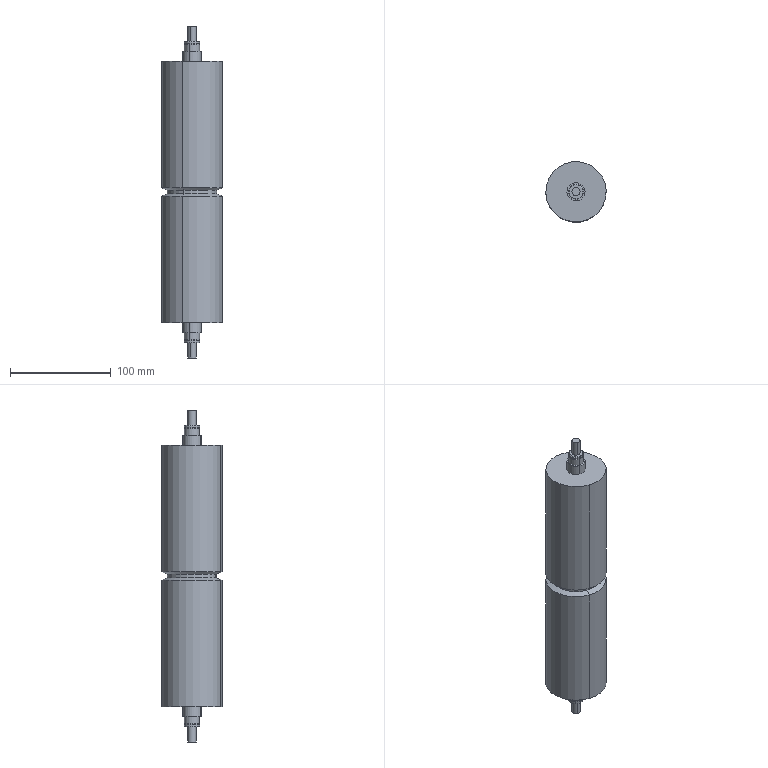Component | SolidWorks | LD101-02--Q1016-Q1-2-1 | 1 solid | 44 faces | box 60 x 60 x 330 mm | volume 739642 mm3 | cylinder 26 | plane 12 | cone 6 | commonest cylinder face diameters 15 x8 8 x4 14.3 x4 60 x4 18 x4 49 x2 | material 45
build123d program:
from build123d import *

# Parameters (mm, degrees)
SKETCH1_R           = 30
SKETCH1_R_2         = 25
EXTRUDE_THIN1_DEPTH = 130
SKETCH10_R          = 30
BOSS_EXTRUDE7_DEPTH = 260
SKETCH2_R           = 30
BOSS_EXTRUDE1_DEPTH = 15
SKETCH3_R           = 9
BOSS_EXTRUDE2_DEPTH = 10
SKETCH5_R           = 7.5
BOSS_EXTRUDE4_DEPTH = 10
BOSS_EXTRUDE5_START = 10
SKETCH6_R           = 7.5
BOSS_EXTRUDE5_DEPTH = 10
CHAMFER4_SIZE       = 0.6
SKETCH7_R           = 4
BOSS_EXTRUDE6_DEPTH = 15
CUT_EXTRUDE1_START  = -3
SKETCH11_OUTSIDE_W  = 130.146
SKETCH11_OUTSIDE_H  = 130.146
SKETCH11_OUTSIDE_R  = 7.15
CUT_EXTRUDE1_DEPTH  = 1.1
CUT_EXTRUDE2_START  = -3
SKETCH12_OUTSIDE_W  = 130.146
SKETCH12_OUTSIDE_H  = 130.146
SKETCH12_OUTSIDE_R  = 7.15
CUT_EXTRUDE2_DEPTH  = 1.1


with BuildPart() as part:
    # Sketch1 → Extrude-Thin1 (new, symmetric)
    with BuildSketch(Plane.XY):
        Circle(SKETCH1_R)
        Circle(SKETCH1_R_2, mode=Mode.SUBTRACT)
    extrude(amount=EXTRUDE_THIN1_DEPTH, both=True)

    # Sketch10 → Boss-Extrude7 (add)
    with BuildSketch(Plane.XY.offset(130)):
        Circle(SKETCH10_R)
    extrude(amount=-BOSS_EXTRUDE7_DEPTH)

    # Sketch2 → Boss-Extrude1 (add)
    with BuildSketch(Plane.XY.offset(130)):
        Circle(SKETCH2_R)
    extrude(amount=-BOSS_EXTRUDE1_DEPTH)

    # Sketch3 → Boss-Extrude2 (add)
    with BuildSketch(Plane.XY.offset(130)):
        Circle(SKETCH3_R)
    extrude(amount=BOSS_EXTRUDE2_DEPTH)

    # Mirror2: part across plane


with BuildPart() as part_1:
    add(part.part)
    add(part.part.mirror(Plane.XY))

    # Sketch5 → Boss-Extrude4 (add)
    with BuildSketch(Plane.XY.offset(140)):
        Circle(SKETCH5_R)
    extrude(amount=BOSS_EXTRUDE4_DEPTH)

    # Sketch6 → Boss-Extrude5 (add)
    with BuildSketch(Plane(origin=(0, 0, -140), x_dir=(-1, 0, 0), z_dir=(0, 0, -1)).offset(BOSS_EXTRUDE5_START)):
        with Locations(Location((0, 0, 0), (0, 0, 180))):
            Circle(SKETCH6_R)
    extrude(amount=-BOSS_EXTRUDE5_DEPTH)

    # Chamfer4
    chamfer4_edges = [part_1.edges().sort_by_distance(p)[0] for p in [
        (-7.5, 0, 150),
    ]]
    chamfer(chamfer4_edges, length=CHAMFER4_SIZE)

    # Sketch7 → Boss-Extrude6 (add)
    with BuildSketch(Plane(origin=(0, 0, -150), x_dir=(-1, 0, 0), z_dir=(0, 0, -1))):
        Circle(SKETCH7_R)
    boss_extrude6 = extrude(amount=BOSS_EXTRUDE6_DEPTH)

    # Mirror3: Boss-Extrude6 across plane
    add(boss_extrude6.mirror(Plane.XY))

    # Sketch8 → Cut-Revolve1 (revolve, cut)
    with BuildSketch(Plane(origin=(0, 0, 0), x_dir=(1, 0, 0), z_dir=(0, 1, 0)), mode=Mode.PRIVATE) as cut_revolve1_sk:
        Polygon((-30, -4), (-30, 4), (-30, 4.025), (-24.5, 1.825), (-24.5, -1.825), (-30, -4.025), align=None)
    revolve(cut_revolve1_sk.sketch.rotate(Axis((0, 0, 70), (0, 0, -1)), 180), axis=Axis((0, 0, 70), (0, 0, -1)), mode=Mode.SUBTRACT)

    # Sketch11 outside → Cut-Extrude1 (cut)
    with BuildSketch(Plane.XY.offset(150).offset(CUT_EXTRUDE1_START)):
        Rectangle(SKETCH11_OUTSIDE_W, SKETCH11_OUTSIDE_H)
        Circle(SKETCH11_OUTSIDE_R, mode=Mode.SUBTRACT)
    extrude(amount=CUT_EXTRUDE1_DEPTH, mode=Mode.SUBTRACT)

    # Sketch12 outside → Cut-Extrude2 (cut)
    with BuildSketch(Plane(origin=(0, 0, -150), x_dir=(-1, 0, 0), z_dir=(0, 0, -1)).offset(CUT_EXTRUDE2_START)):
        Rectangle(SKETCH12_OUTSIDE_W, SKETCH12_OUTSIDE_H)
        with Locations(Location((0, 0, 0), (0, 0, 180))):
            Circle(SKETCH12_OUTSIDE_R, mode=Mode.SUBTRACT)
    extrude(amount=CUT_EXTRUDE2_DEPTH, mode=Mode.SUBTRACT)


solid = part_1.part

# Placed as in the assembly
solid = solid.moved(Location((121.71, -181.897, 146.257), (0, 0, 0)))